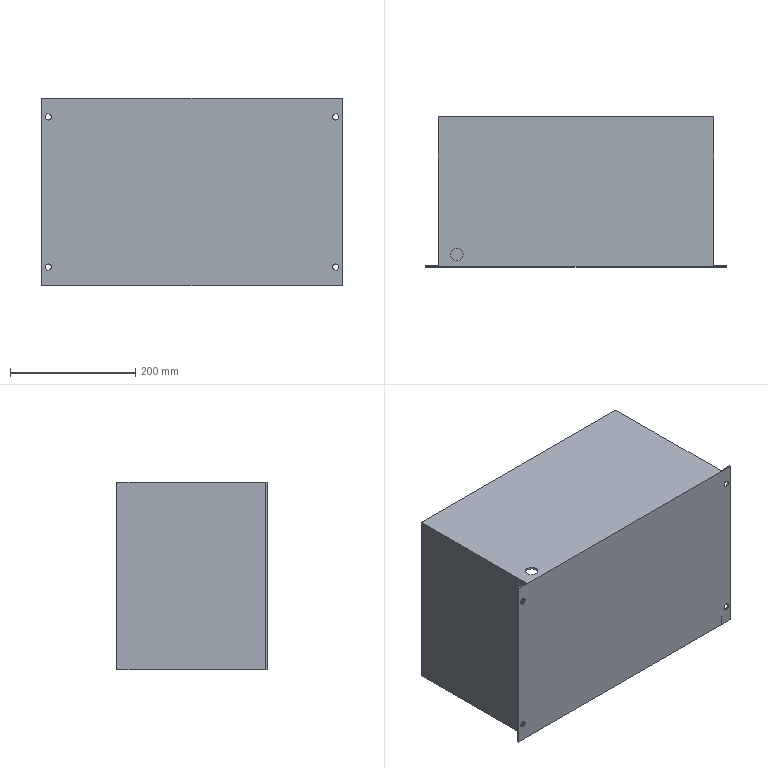Component | SolidWorks | FuelTank-1_FuelTank-1 | 1 solid | 43 faces | box 480 x 240 x 300 mm | volume 1516909 mm3 | plane 25 | cylinder 18 | commonest cylinder face diameters 7 x8 10 x8 20 x2
build123d program:
from build123d import *

# Parameters (mm, degrees)
SKETCH1_W           = 440
SKETCH1_H           = 240
BOSS_EXTRUDE1_DEPTH = 300
SHELL1_T            = -3
SKETCH2_W           = 434
SKETCH2_H           = 294
SKETCH2_W_2         = 394
SKETCH2_H_2         = 254
EXTRUDE_THIN1_DEPTH = 2
SKETCH3_W           = 20
SKETCH3_H           = 2
BOSS_EXTRUDE2_DEPTH = 300
SKETCH4_R           = 5
CUT_EXTRUDE1_DEPTH  = 2
SKETCH5_R           = 3.5
CUT_EXTRUDE2_DEPTH  = 3
SKETCH6_R           = 10
CUT_EXTRUDE3_DEPTH  = 3


with BuildPart() as part:
    # Sketch1 → Boss-Extrude1 (new body)
    with BuildSketch(Plane.XY):
        with Locations((153.598, -88.271)):
            Rectangle(SKETCH1_W, SKETCH1_H)
    extrude(amount=BOSS_EXTRUDE1_DEPTH)

    # Shell1
    shell1_openings = [part.faces().sort_by_distance(p)[0] for p in [
        (153.598, 31.729, 150),
    ]]
    offset(amount=SHELL1_T, openings=shell1_openings, kind=Kind.INTERSECTION)

    # Sketch2 → Extrude-Thin1 (add)
    with BuildSketch(Plane(origin=(0, 28.729, 0), x_dir=(1, 0, 0), z_dir=(0, 1, 0))):
        with Locations((153.598, -150)):
            Rectangle(SKETCH2_W, SKETCH2_H)
        with Locations((153.598, -150)):
            Rectangle(SKETCH2_W_2, SKETCH2_H_2, mode=Mode.SUBTRACT)
    extrude(amount=-EXTRUDE_THIN1_DEPTH)

    # Sketch3 → Boss-Extrude2 (add)
    with BuildSketch(Plane.XY.offset(300)):
        with Locations((383.598, -207.271)):
            Rectangle(SKETCH3_W, SKETCH3_H)
        with Locations((-76.402, -207.271)):
            Rectangle(SKETCH3_W, SKETCH3_H)
    extrude(amount=-BOSS_EXTRUDE2_DEPTH)

    # Sketch4 → Cut-Extrude1 (cut)
    with BuildSketch(Plane(origin=(0, -206.271, 0), x_dir=(1, 0, 0), z_dir=(0, 1, 0))):
        with Locations(Location((383.598, -30, 0), (0, 0, 270))):
            Circle(SKETCH4_R)
        with Locations(Location((383.598, -270, 0), (0, 0, 270))):
            Circle(SKETCH4_R)
        with Locations(Location((-76.402, -30, 0), (0, 0, 270))):
            Circle(SKETCH4_R)
        with Locations(Location((-76.402, -270, 0), (0, 0, 270))):
            Circle(SKETCH4_R)
    extrude(amount=-CUT_EXTRUDE1_DEPTH, mode=Mode.SUBTRACT)

    # Sketch5 → Cut-Extrude2 (cut)
    with BuildSketch(Plane(origin=(0, 28.729, 0), x_dir=(1, 0, 0), z_dir=(0, 1, 0))):
        with Locations(Location((359.598, -14, 0), (0, 0, 270))):
            Circle(SKETCH5_R)
        with Locations(Location((359.598, -286, 0), (0, 0, 270))):
            Circle(SKETCH5_R)
        with Locations(Location((-52.402, -286, 0), (0, 0, 270))):
            Circle(SKETCH5_R)
        with Locations(Location((-52.402, -14, 0), (0, 0, 270))):
            Circle(SKETCH5_R)
    extrude(amount=-CUT_EXTRUDE2_DEPTH, mode=Mode.SUBTRACT)

    # Sketch6 → Cut-Extrude3 (cut)
    with BuildSketch(Plane.XY.offset(300)):
        with Locations((-36.842, -188.502)):
            Circle(SKETCH6_R)
    extrude(amount=-CUT_EXTRUDE3_DEPTH, mode=Mode.SUBTRACT)


solid = part.part

# Placed as in the assembly
solid = solid.moved(Location((31.852, -500.162, -671.519), (0, 0, 0)))